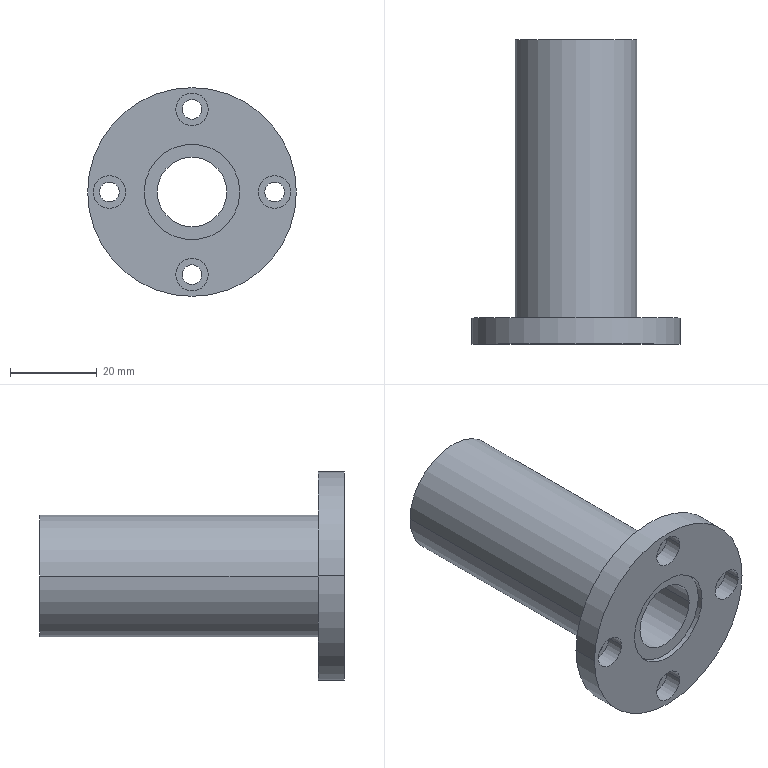Component | SolidWorks | SL021-1RoundFlangeExtendedType-416.SL4PRT-4 | 1 solid | 35 faces | box 48 x 70 x 48 mm | volume 34916 mm3 | cylinder 26 | plane 9 | commonest cylinder face diameters 4.5 x8 7.5 x8 22 x4 28 x2 48 x2 16 x2 | material Q235
STEP:
#1=COLOUR_RGB('',0.7922,0.8196,0.9333);
#2=FILL_AREA_STYLE_COLOUR('',#1);
#3=FILL_AREA_STYLE('',(#2));
#4=SURFACE_STYLE_FILL_AREA(#3);
#5=SURFACE_SIDE_STYLE('',(#4));
#6=SURFACE_STYLE_USAGE(.BOTH.,#5);
#7=PRESENTATION_STYLE_ASSIGNMENT((#6));
#8=CARTESIAN_POINT('',(-2.762,-0.807,0.1426));
#9=VERTEX_POINT('',#8);
#10=CARTESIAN_POINT('',(-1.66,-0.807,0.1426));
#11=VERTEX_POINT('',#10);
#12=CARTESIAN_POINT('',(-2.211,-0.807,0.1426));
#13=DIRECTION('',(-0.,1.,-0.));
#14=DIRECTION('',(-1.,0.,0.));
#15=AXIS2_PLACEMENT_3D('',#12,#13,#14);
#16=CIRCLE('',#15,0.5512);
#17=EDGE_CURVE('',#9,#11,#16,.T.);
#18=ORIENTED_EDGE('',*,*,#17,.T.);
#19=CARTESIAN_POINT('',(-1.66,1.713,0.1426));
#20=VERTEX_POINT('',#19);
#21=CARTESIAN_POINT('',(-1.66,1.713,0.1426));
#22=DIRECTION('',(-0.,1.,-0.));
#23=VECTOR('',#22,39.37);
#24=LINE('',#21,#23);
#25=EDGE_CURVE('',#11,#20,#24,.T.);
#26=ORIENTED_EDGE('',*,*,#25,.T.);
#27=CARTESIAN_POINT('',(-2.762,1.713,0.1426));
#28=VERTEX_POINT('',#27);
#29=CARTESIAN_POINT('',(-2.211,1.713,0.1426));
#30=DIRECTION('',(0.,-1.,0.));
#31=DIRECTION('',(-1.,0.,0.));
#32=AXIS2_PLACEMENT_3D('',#29,#30,#31);
#33=CIRCLE('',#32,0.5512);
#34=EDGE_CURVE('',#20,#28,#33,.T.);
#35=ORIENTED_EDGE('',*,*,#34,.T.);
#36=CARTESIAN_POINT('',(-2.762,1.713,0.1426));
#37=DIRECTION('',(-0.,1.,-0.));
#38=VECTOR('',#37,39.37);
#39=LINE('',#36,#38);
#40=EDGE_CURVE('',#9,#28,#39,.T.);
#41=ORIENTED_EDGE('',*,*,#40,.F.);
#42=EDGE_LOOP('',(#18,#26,#35,#41));
#43=FACE_OUTER_BOUND('',#42,.T.);
#44=CARTESIAN_POINT('',(-2.211,1.713,0.1426));
#45=DIRECTION('',(-0.,1.,-0.));
#46=DIRECTION('',(-1.,0.,0.));
#47=AXIS2_PLACEMENT_3D('',#44,#45,#46);
#48=CYLINDRICAL_SURFACE('',#47,0.5512);
#49=ADVANCED_FACE('',(#43),#48,.T.);
#50=CARTESIAN_POINT('',(-1.778,1.665,0.1426));
#51=VERTEX_POINT('',#50);
#52=CARTESIAN_POINT('',(-2.644,1.665,0.1426));
#53=VERTEX_POINT('',#52);
#54=CARTESIAN_POINT('',(-2.211,1.665,0.1426));
#55=DIRECTION('',(-0.,1.,-0.));
#56=DIRECTION('',(-1.,0.,0.));
#57=AXIS2_PLACEMENT_3D('',#54,#55,#56);
#58=CIRCLE('',#57,0.4331);
#59=EDGE_CURVE('',#51,#53,#58,.T.);
#60=ORIENTED_EDGE('',*,*,#59,.F.);
#61=CARTESIAN_POINT('',(-1.778,1.713,0.1426));
#62=VERTEX_POINT('',#61);
#63=CARTESIAN_POINT('',(-1.778,1.713,0.1426));
#64=DIRECTION('',(-0.,1.,-0.));
#65=VECTOR('',#64,39.37);
#66=LINE('',#63,#65);
#67=EDGE_CURVE('',#51,#62,#66,.T.);
#68=ORIENTED_EDGE('',*,*,#67,.T.);
#69=CARTESIAN_POINT('',(-2.644,1.713,0.1426));
#70=VERTEX_POINT('',#69);
#71=CARTESIAN_POINT('',(-2.211,1.713,0.1426));
#72=DIRECTION('',(0.,-1.,0.));
#73=DIRECTION('',(-1.,0.,0.));
#74=AXIS2_PLACEMENT_3D('',#71,#72,#73);
#75=CIRCLE('',#74,0.4331);
#76=EDGE_CURVE('',#70,#62,#75,.T.);
#77=ORIENTED_EDGE('',*,*,#76,.F.);
#78=CARTESIAN_POINT('',(-2.644,1.713,0.1426));
#79=DIRECTION('',(-0.,1.,-0.));
#80=VECTOR('',#79,39.37);
#81=LINE('',#78,#80);
#82=EDGE_CURVE('',#53,#70,#81,.T.);
#83=ORIENTED_EDGE('',*,*,#82,.F.);
#84=EDGE_LOOP('',(#60,#68,#77,#83));
#85=FACE_OUTER_BOUND('',#84,.T.);
#86=CARTESIAN_POINT('',(-2.211,1.713,0.1426));
#87=DIRECTION('',(-0.,1.,-0.));
#88=DIRECTION('',(-1.,0.,0.));
#89=AXIS2_PLACEMENT_3D('',#86,#87,#88);
#90=CYLINDRICAL_SURFACE('',#89,0.4331);
#91=ADVANCED_FACE('',(#85),#90,.F.);
#92=CARTESIAN_POINT('',(-3.156,-1.043,0.1426));
#93=VERTEX_POINT('',#92);
#94=CARTESIAN_POINT('',(-1.266,-1.043,0.1426));
#95=VERTEX_POINT('',#94);
#96=CARTESIAN_POINT('',(-2.211,-1.043,0.1426));
#97=DIRECTION('',(-0.,1.,-0.));
#98=DIRECTION('',(-1.,0.,0.));
#99=AXIS2_PLACEMENT_3D('',#96,#97,#98);
#100=CIRCLE('',#99,0.9449);
#101=EDGE_CURVE('',#93,#95,#100,.T.);
#102=ORIENTED_EDGE('',*,*,#101,.T.);
#103=CARTESIAN_POINT('',(-1.266,-0.807,0.1426));
#104=VERTEX_POINT('',#103);
#105=CARTESIAN_POINT('',(-1.266,1.713,0.1426));
#106=DIRECTION('',(-0.,1.,-0.));
#107=VECTOR('',#106,39.37);
#108=LINE('',#105,#107);
#109=EDGE_CURVE('',#95,#104,#108,.T.);
#110=ORIENTED_EDGE('',*,*,#109,.T.);
#111=CARTESIAN_POINT('',(-3.156,-0.807,0.1426));
#112=VERTEX_POINT('',#111);
#113=CARTESIAN_POINT('',(-2.211,-0.807,0.1426));
#114=DIRECTION('',(-0.,1.,-0.));
#115=DIRECTION('',(-1.,0.,0.));
#116=AXIS2_PLACEMENT_3D('',#113,#114,#115);
#117=CIRCLE('',#116,0.9449);
#118=EDGE_CURVE('',#112,#104,#117,.T.);
#119=ORIENTED_EDGE('',*,*,#118,.F.);
#120=CARTESIAN_POINT('',(-3.156,1.713,0.1426));
#121=DIRECTION('',(-0.,1.,-0.));
#122=VECTOR('',#121,39.37);
#123=LINE('',#120,#122);
#124=EDGE_CURVE('',#93,#112,#123,.T.);
#125=ORIENTED_EDGE('',*,*,#124,.F.);
#126=EDGE_LOOP('',(#102,#110,#119,#125));
#127=FACE_OUTER_BOUND('',#126,.T.);
#128=CARTESIAN_POINT('',(-2.211,1.713,0.1426));
#129=DIRECTION('',(-0.,1.,-0.));
#130=DIRECTION('',(-1.,0.,0.));
#131=AXIS2_PLACEMENT_3D('',#128,#129,#130);
#132=CYLINDRICAL_SURFACE('',#131,0.9449);
#133=ADVANCED_FACE('',(#127),#132,.T.);
#134=CARTESIAN_POINT('',(-2.3,-0.807,0.8906));
#135=VERTEX_POINT('',#134);
#136=CARTESIAN_POINT('',(-2.123,-0.807,0.8906));
#137=VERTEX_POINT('',#136);
#138=CARTESIAN_POINT('',(-2.211,-0.807,0.8906));
#139=DIRECTION('',(0.,-1.,0.));
#140=DIRECTION('',(1.,0.,0.));
#141=AXIS2_PLACEMENT_3D('',#138,#139,#140);
#142=CIRCLE('',#141,0.08858);
#143=EDGE_CURVE('',#135,#137,#142,.T.);
#144=ORIENTED_EDGE('',*,*,#143,.F.);
#145=CARTESIAN_POINT('',(-2.3,-0.8819,0.8906));
#146=VERTEX_POINT('',#145);
#147=CARTESIAN_POINT('',(-2.3,1.713,0.8906));
#148=DIRECTION('',(0.,-1.,0.));
#149=VECTOR('',#148,39.37);
#150=LINE('',#147,#149);
#151=EDGE_CURVE('',#135,#146,#150,.T.);
#152=ORIENTED_EDGE('',*,*,#151,.T.);
#153=CARTESIAN_POINT('',(-2.123,-0.8819,0.8906));
#154=VERTEX_POINT('',#153);
#155=CARTESIAN_POINT('',(-2.211,-0.8819,0.8906));
#156=DIRECTION('',(-0.,1.,-0.));
#157=DIRECTION('',(1.,0.,0.));
#158=AXIS2_PLACEMENT_3D('',#155,#156,#157);
#159=CIRCLE('',#158,0.08858);
#160=EDGE_CURVE('',#154,#146,#159,.T.);
#161=ORIENTED_EDGE('',*,*,#160,.F.);
#162=CARTESIAN_POINT('',(-2.123,1.713,0.8906));
#163=DIRECTION('',(0.,-1.,0.));
#164=VECTOR('',#163,39.37);
#165=LINE('',#162,#164);
#166=EDGE_CURVE('',#137,#154,#165,.T.);
#167=ORIENTED_EDGE('',*,*,#166,.F.);
#168=EDGE_LOOP('',(#144,#152,#161,#167));
#169=FACE_OUTER_BOUND('',#168,.T.);
#170=CARTESIAN_POINT('',(-2.211,1.713,0.8906));
#171=DIRECTION('',(0.,-1.,0.));
#172=DIRECTION('',(1.,0.,0.));
#173=AXIS2_PLACEMENT_3D('',#170,#171,#172);
#174=CYLINDRICAL_SURFACE('',#173,0.08858);
#175=ADVANCED_FACE('',(#169),#174,.F.);
#176=CARTESIAN_POINT('',(-1.552,-0.807,0.1426));
#177=VERTEX_POINT('',#176);
#178=CARTESIAN_POINT('',(-1.375,-0.807,0.1426));
#179=VERTEX_POINT('',#178);
#180=CARTESIAN_POINT('',(-1.463,-0.807,0.1426));
#181=DIRECTION('',(0.,-1.,0.));
#182=DIRECTION('',(1.,0.,-0.));
#183=AXIS2_PLACEMENT_3D('',#180,#181,#182);
#184=CIRCLE('',#183,0.08858);
#185=EDGE_CURVE('',#177,#179,#184,.T.);
#186=ORIENTED_EDGE('',*,*,#185,.F.);
#187=CARTESIAN_POINT('',(-1.552,-0.8819,0.1426));
#188=VERTEX_POINT('',#187);
#189=CARTESIAN_POINT('',(-1.552,1.713,0.1426));
#190=DIRECTION('',(0.,-1.,0.));
#191=VECTOR('',#190,39.37);
#192=LINE('',#189,#191);
#193=EDGE_CURVE('',#177,#188,#192,.T.);
#194=ORIENTED_EDGE('',*,*,#193,.T.);
#195=CARTESIAN_POINT('',(-1.375,-0.8819,0.1426));
#196=VERTEX_POINT('',#195);
#197=CARTESIAN_POINT('',(-1.463,-0.8819,0.1426));
#198=DIRECTION('',(-0.,1.,-0.));
#199=DIRECTION('',(1.,0.,-0.));
#200=AXIS2_PLACEMENT_3D('',#197,#198,#199);
#201=CIRCLE('',#200,0.08858);
#202=EDGE_CURVE('',#196,#188,#201,.T.);
#203=ORIENTED_EDGE('',*,*,#202,.F.);
#204=CARTESIAN_POINT('',(-1.375,1.713,0.1426));
#205=DIRECTION('',(0.,-1.,0.));
#206=VECTOR('',#205,39.37);
#207=LINE('',#204,#206);
#208=EDGE_CURVE('',#179,#196,#207,.T.);
#209=ORIENTED_EDGE('',*,*,#208,.F.);
#210=EDGE_LOOP('',(#186,#194,#203,#209));
#211=FACE_OUTER_BOUND('',#210,.T.);
#212=CARTESIAN_POINT('',(-1.463,1.713,0.1426));
#213=DIRECTION('',(0.,-1.,0.));
#214=DIRECTION('',(1.,0.,-0.));
#215=AXIS2_PLACEMENT_3D('',#212,#213,#214);
#216=CYLINDRICAL_SURFACE('',#215,0.08858);
#217=ADVANCED_FACE('',(#211),#216,.F.);
#218=CARTESIAN_POINT('',(-2.3,-0.807,-0.6054));
#219=VERTEX_POINT('',#218);
#220=CARTESIAN_POINT('',(-2.123,-0.807,-0.6054));
#221=VERTEX_POINT('',#220);
#222=CARTESIAN_POINT('',(-2.211,-0.807,-0.6054));
#223=DIRECTION('',(0.,-1.,0.));
#224=DIRECTION('',(1.,0.,0.));
#225=AXIS2_PLACEMENT_3D('',#222,#223,#224);
#226=CIRCLE('',#225,0.08858);
#227=EDGE_CURVE('',#219,#221,#226,.T.);
#228=ORIENTED_EDGE('',*,*,#227,.F.);
#229=CARTESIAN_POINT('',(-2.3,-0.8819,-0.6054));
#230=VERTEX_POINT('',#229);
#231=CARTESIAN_POINT('',(-2.3,1.713,-0.6054));
#232=DIRECTION('',(0.,-1.,0.));
#233=VECTOR('',#232,39.37);
#234=LINE('',#231,#233);
#235=EDGE_CURVE('',#219,#230,#234,.T.);
#236=ORIENTED_EDGE('',*,*,#235,.T.);
#237=CARTESIAN_POINT('',(-2.123,-0.8819,-0.6054));
#238=VERTEX_POINT('',#237);
#239=CARTESIAN_POINT('',(-2.211,-0.8819,-0.6054));
#240=DIRECTION('',(-0.,1.,-0.));
#241=DIRECTION('',(1.,0.,0.));
#242=AXIS2_PLACEMENT_3D('',#239,#240,#241);
#243=CIRCLE('',#242,0.08858);
#244=EDGE_CURVE('',#238,#230,#243,.T.);
#245=ORIENTED_EDGE('',*,*,#244,.F.);
#246=CARTESIAN_POINT('',(-2.123,1.713,-0.6054));
#247=DIRECTION('',(0.,-1.,0.));
#248=VECTOR('',#247,39.37);
#249=LINE('',#246,#248);
#250=EDGE_CURVE('',#221,#238,#249,.T.);
#251=ORIENTED_EDGE('',*,*,#250,.F.);
#252=EDGE_LOOP('',(#228,#236,#245,#251));
#253=FACE_OUTER_BOUND('',#252,.T.);
#254=CARTESIAN_POINT('',(-2.211,1.713,-0.6054));
#255=DIRECTION('',(0.,-1.,0.));
#256=DIRECTION('',(1.,0.,0.));
#257=AXIS2_PLACEMENT_3D('',#254,#255,#256);
#258=CYLINDRICAL_SURFACE('',#257,0.08858);
#259=ADVANCED_FACE('',(#253),#258,.F.);
#260=CARTESIAN_POINT('',(-3.048,-0.807,0.1426));
#261=VERTEX_POINT('',#260);
#262=CARTESIAN_POINT('',(-2.871,-0.807,0.1426));
#263=VERTEX_POINT('',#262);
#264=CARTESIAN_POINT('',(-2.959,-0.807,0.1426));
#265=DIRECTION('',(0.,-1.,0.));
#266=DIRECTION('',(1.,0.,-0.));
#267=AXIS2_PLACEMENT_3D('',#264,#265,#266);
#268=CIRCLE('',#267,0.08858);
#269=EDGE_CURVE('',#261,#263,#268,.T.);
#270=ORIENTED_EDGE('',*,*,#269,.F.);
#271=CARTESIAN_POINT('',(-3.048,-0.8819,0.1426));
#272=VERTEX_POINT('',#271);
#273=CARTESIAN_POINT('',(-3.048,1.713,0.1426));
#274=DIRECTION('',(0.,-1.,0.));
#275=VECTOR('',#274,39.37);
#276=LINE('',#273,#275);
#277=EDGE_CURVE('',#261,#272,#276,.T.);
#278=ORIENTED_EDGE('',*,*,#277,.T.);
#279=CARTESIAN_POINT('',(-2.871,-0.8819,0.1426));
#280=VERTEX_POINT('',#279);
#281=CARTESIAN_POINT('',(-2.959,-0.8819,0.1426));
#282=DIRECTION('',(-0.,1.,-0.));
#283=DIRECTION('',(1.,0.,-0.));
#284=AXIS2_PLACEMENT_3D('',#281,#282,#283);
#285=CIRCLE('',#284,0.08858);
#286=EDGE_CURVE('',#280,#272,#285,.T.);
#287=ORIENTED_EDGE('',*,*,#286,.F.);
#288=CARTESIAN_POINT('',(-2.871,1.713,0.1426));
#289=DIRECTION('',(0.,-1.,0.));
#290=VECTOR('',#289,39.37);
#291=LINE('',#288,#290);
#292=EDGE_CURVE('',#263,#280,#291,.T.);
#293=ORIENTED_EDGE('',*,*,#292,.F.);
#294=EDGE_LOOP('',(#270,#278,#287,#293));
#295=FACE_OUTER_BOUND('',#294,.T.);
#296=CARTESIAN_POINT('',(-2.959,1.713,0.1426));
#297=DIRECTION('',(0.,-1.,0.));
#298=DIRECTION('',(1.,0.,-0.));
#299=AXIS2_PLACEMENT_3D('',#296,#297,#298);
#300=CYLINDRICAL_SURFACE('',#299,0.08858);
#301=ADVANCED_FACE('',(#295),#300,.F.);
#302=CARTESIAN_POINT('',(-1.896,-0.996,0.1426));
#303=VERTEX_POINT('',#302);
#304=CARTESIAN_POINT('',(-2.526,-0.996,0.1426));
#305=VERTEX_POINT('',#304);
#306=CARTESIAN_POINT('',(-2.211,-0.996,0.1426));
#307=DIRECTION('',(-0.,1.,-0.));
#308=DIRECTION('',(-1.,0.,0.));
#309=AXIS2_PLACEMENT_3D('',#306,#307,#308);
#310=CIRCLE('',#309,0.315);
#311=EDGE_CURVE('',#303,#305,#310,.T.);
#312=ORIENTED_EDGE('',*,*,#311,.F.);
#313=CARTESIAN_POINT('',(-1.896,1.665,0.1426));
#314=VERTEX_POINT('',#313);
#315=CARTESIAN_POINT('',(-1.896,1.713,0.1426));
#316=DIRECTION('',(-0.,1.,-0.));
#317=VECTOR('',#316,39.37);
#318=LINE('',#315,#317);
#319=EDGE_CURVE('',#303,#314,#318,.T.);
#320=ORIENTED_EDGE('',*,*,#319,.T.);
#321=CARTESIAN_POINT('',(-2.526,1.665,0.1426));
#322=VERTEX_POINT('',#321);
#323=CARTESIAN_POINT('',(-2.211,1.665,0.1426));
#324=DIRECTION('',(-0.,1.,-0.));
#325=DIRECTION('',(-1.,0.,0.));
#326=AXIS2_PLACEMENT_3D('',#323,#324,#325);
#327=CIRCLE('',#326,0.315);
#328=EDGE_CURVE('',#314,#322,#327,.T.);
#329=ORIENTED_EDGE('',*,*,#328,.T.);
#330=CARTESIAN_POINT('',(-2.526,1.713,0.1426));
#331=DIRECTION('',(-0.,1.,-0.));
#332=VECTOR('',#331,39.37);
#333=LINE('',#330,#332);
#334=EDGE_CURVE('',#305,#322,#333,.T.);
#335=ORIENTED_EDGE('',*,*,#334,.F.);
#336=EDGE_LOOP('',(#312,#320,#329,#335));
#337=FACE_OUTER_BOUND('',#336,.T.);
#338=CARTESIAN_POINT('',(-2.211,1.713,0.1426));
#339=DIRECTION('',(-0.,1.,-0.));
#340=DIRECTION('',(-1.,0.,0.));
#341=AXIS2_PLACEMENT_3D('',#338,#339,#340);
#342=CYLINDRICAL_SURFACE('',#341,0.315);
#343=ADVANCED_FACE('',(#337),#342,.F.);
#344=CARTESIAN_POINT('',(-1.778,-1.043,0.1426));
#345=VERTEX_POINT('',#344);
#346=CARTESIAN_POINT('',(-2.644,-1.043,0.1426));
#347=VERTEX_POINT('',#346);
#348=CARTESIAN_POINT('',(-2.211,-1.043,0.1426));
#349=DIRECTION('',(-0.,1.,-0.));
#350=DIRECTION('',(-1.,0.,0.));
#351=AXIS2_PLACEMENT_3D('',#348,#349,#350);
#352=CIRCLE('',#351,0.4331);
#353=EDGE_CURVE('',#345,#347,#352,.T.);
#354=ORIENTED_EDGE('',*,*,#353,.F.);
#355=CARTESIAN_POINT('',(-1.778,-0.996,0.1426));
#356=VERTEX_POINT('',#355);
#357=CARTESIAN_POINT('',(-1.778,1.713,0.1426));
#358=DIRECTION('',(-0.,1.,-0.));
#359=VECTOR('',#358,39.37);
#360=LINE('',#357,#359);
#361=EDGE_CURVE('',#345,#356,#360,.T.);
#362=ORIENTED_EDGE('',*,*,#361,.T.);
#363=CARTESIAN_POINT('',(-2.644,-0.996,0.1426));
#364=VERTEX_POINT('',#363);
#365=CARTESIAN_POINT('',(-2.211,-0.996,0.1426));
#366=DIRECTION('',(0.,-1.,0.));
#367=DIRECTION('',(-1.,0.,0.));
#368=AXIS2_PLACEMENT_3D('',#365,#366,#367);
#369=CIRCLE('',#368,0.4331);
#370=EDGE_CURVE('',#364,#356,#369,.T.);
#371=ORIENTED_EDGE('',*,*,#370,.F.);
#372=CARTESIAN_POINT('',(-2.644,1.713,0.1426));
#373=DIRECTION('',(-0.,1.,-0.));
#374=VECTOR('',#373,39.37);
#375=LINE('',#372,#374);
#376=EDGE_CURVE('',#347,#364,#375,.T.);
#377=ORIENTED_EDGE('',*,*,#376,.F.);
#378=EDGE_LOOP('',(#354,#362,#371,#377));
#379=FACE_OUTER_BOUND('',#378,.T.);
#380=CARTESIAN_POINT('',(-2.211,1.713,0.1426));
#381=DIRECTION('',(-0.,1.,-0.));
#382=DIRECTION('',(-1.,0.,0.));
#383=AXIS2_PLACEMENT_3D('',#380,#381,#382);
#384=CYLINDRICAL_SURFACE('',#383,0.4331);
#385=ADVANCED_FACE('',(#379),#384,.F.);
#386=CARTESIAN_POINT('',(-2.359,-0.8819,0.8906));
#387=VERTEX_POINT('',#386);
#388=CARTESIAN_POINT('',(-2.064,-0.8819,0.8906));
#389=VERTEX_POINT('',#388);
#390=CARTESIAN_POINT('',(-2.211,-0.8819,0.8906));
#391=DIRECTION('',(0.,-1.,0.));
#392=DIRECTION('',(1.,0.,0.));
#393=AXIS2_PLACEMENT_3D('',#390,#391,#392);
#394=CIRCLE('',#393,0.1476);
#395=EDGE_CURVE('',#387,#389,#394,.T.);
#396=ORIENTED_EDGE('',*,*,#395,.F.);
#397=CARTESIAN_POINT('',(-2.359,-1.043,0.8906));
#398=VERTEX_POINT('',#397);
#399=CARTESIAN_POINT('',(-2.359,-0.8819,0.8906));
#400=DIRECTION('',(0.,-1.,0.));
#401=VECTOR('',#400,39.37);
#402=LINE('',#399,#401);
#403=EDGE_CURVE('',#387,#398,#402,.T.);
#404=ORIENTED_EDGE('',*,*,#403,.T.);
#405=CARTESIAN_POINT('',(-2.064,-1.043,0.8906));
#406=VERTEX_POINT('',#405);
#407=CARTESIAN_POINT('',(-2.211,-1.043,0.8906));
#408=DIRECTION('',(-0.,1.,-0.));
#409=DIRECTION('',(1.,0.,0.));
#410=AXIS2_PLACEMENT_3D('',#407,#408,#409);
#411=CIRCLE('',#410,0.1476);
#412=EDGE_CURVE('',#406,#398,#411,.T.);
#413=ORIENTED_EDGE('',*,*,#412,.F.);
#414=CARTESIAN_POINT('',(-2.064,-0.8819,0.8906));
#415=DIRECTION('',(0.,-1.,0.));
#416=VECTOR('',#415,39.37);
#417=LINE('',#414,#416);
#418=EDGE_CURVE('',#389,#406,#417,.T.);
#419=ORIENTED_EDGE('',*,*,#418,.F.);
#420=EDGE_LOOP('',(#396,#404,#413,#419));
#421=FACE_OUTER_BOUND('',#420,.T.);
#422=CARTESIAN_POINT('',(-2.211,-0.8819,0.8906));
#423=DIRECTION('',(0.,-1.,0.));
#424=DIRECTION('',(1.,0.,0.));
#425=AXIS2_PLACEMENT_3D('',#422,#423,#424);
#426=CYLINDRICAL_SURFACE('',#425,0.1476);
#427=ADVANCED_FACE('',(#421),#426,.F.);
#428=CARTESIAN_POINT('',(-1.611,-0.8819,0.1426));
#429=VERTEX_POINT('',#428);
#430=CARTESIAN_POINT('',(-1.315,-0.8819,0.1426));
#431=VERTEX_POINT('',#430);
#432=CARTESIAN_POINT('',(-1.463,-0.8819,0.1426));
#433=DIRECTION('',(0.,-1.,0.));
#434=DIRECTION('',(1.,0.,-0.));
#435=AXIS2_PLACEMENT_3D('',#432,#433,#434);
#436=CIRCLE('',#435,0.1476);
#437=EDGE_CURVE('',#429,#431,#436,.T.);
#438=ORIENTED_EDGE('',*,*,#437,.F.);
#439=CARTESIAN_POINT('',(-1.611,-1.043,0.1426));
#440=VERTEX_POINT('',#439);
#441=CARTESIAN_POINT('',(-1.611,-0.8819,0.1426));
#442=DIRECTION('',(0.,-1.,0.));
#443=VECTOR('',#442,39.37);
#444=LINE('',#441,#443);
#445=EDGE_CURVE('',#429,#440,#444,.T.);
#446=ORIENTED_EDGE('',*,*,#445,.T.);
#447=CARTESIAN_POINT('',(-1.315,-1.043,0.1426));
#448=VERTEX_POINT('',#447);
#449=CARTESIAN_POINT('',(-1.463,-1.043,0.1426));
#450=DIRECTION('',(-0.,1.,-0.));
#451=DIRECTION('',(1.,0.,-0.));
#452=AXIS2_PLACEMENT_3D('',#449,#450,#451);
#453=CIRCLE('',#452,0.1476);
#454=EDGE_CURVE('',#448,#440,#453,.T.);
#455=ORIENTED_EDGE('',*,*,#454,.F.);
#456=CARTESIAN_POINT('',(-1.315,-0.8819,0.1426));
#457=DIRECTION('',(0.,-1.,0.));
#458=VECTOR('',#457,39.37);
#459=LINE('',#456,#458);
#460=EDGE_CURVE('',#431,#448,#459,.T.);
#461=ORIENTED_EDGE('',*,*,#460,.F.);
#462=EDGE_LOOP('',(#438,#446,#455,#461));
#463=FACE_OUTER_BOUND('',#462,.T.);
#464=CARTESIAN_POINT('',(-1.463,-0.8819,0.1426));
#465=DIRECTION('',(0.,-1.,0.));
#466=DIRECTION('',(1.,0.,-0.));
#467=AXIS2_PLACEMENT_3D('',#464,#465,#466);
#468=CYLINDRICAL_SURFACE('',#467,0.1476);
#469=ADVANCED_FACE('',(#463),#468,.F.);
#470=CARTESIAN_POINT('',(-2.359,-0.8819,-0.6054));
#471=VERTEX_POINT('',#470);
#472=CARTESIAN_POINT('',(-2.064,-0.8819,-0.6054));
#473=VERTEX_POINT('',#472);
#474=CARTESIAN_POINT('',(-2.211,-0.8819,-0.6054));
#475=DIRECTION('',(0.,-1.,0.));
#476=DIRECTION('',(1.,0.,0.));
#477=AXIS2_PLACEMENT_3D('',#474,#475,#476);
#478=CIRCLE('',#477,0.1476);
#479=EDGE_CURVE('',#471,#473,#478,.T.);
#480=ORIENTED_EDGE('',*,*,#479,.F.);
#481=CARTESIAN_POINT('',(-2.359,-1.043,-0.6054));
#482=VERTEX_POINT('',#481);
#483=CARTESIAN_POINT('',(-2.359,-0.8819,-0.6054));
#484=DIRECTION('',(0.,-1.,0.));
#485=VECTOR('',#484,39.37);
#486=LINE('',#483,#485);
#487=EDGE_CURVE('',#471,#482,#486,.T.);
#488=ORIENTED_EDGE('',*,*,#487,.T.);
#489=CARTESIAN_POINT('',(-2.064,-1.043,-0.6054));
#490=VERTEX_POINT('',#489);
#491=CARTESIAN_POINT('',(-2.211,-1.043,-0.6054));
#492=DIRECTION('',(-0.,1.,-0.));
#493=DIRECTION('',(1.,0.,0.));
#494=AXIS2_PLACEMENT_3D('',#491,#492,#493);
#495=CIRCLE('',#494,0.1476);
#496=EDGE_CURVE('',#490,#482,#495,.T.);
#497=ORIENTED_EDGE('',*,*,#496,.F.);
#498=CARTESIAN_POINT('',(-2.064,-0.8819,-0.6054));
#499=DIRECTION('',(0.,-1.,0.));
#500=VECTOR('',#499,39.37);
#501=LINE('',#498,#500);
#502=EDGE_CURVE('',#473,#490,#501,.T.);
#503=ORIENTED_EDGE('',*,*,#502,.F.);
#504=EDGE_LOOP('',(#480,#488,#497,#503));
#505=FACE_OUTER_BOUND('',#504,.T.);
#506=CARTESIAN_POINT('',(-2.211,-0.8819,-0.6054));
#507=DIRECTION('',(0.,-1.,0.));
#508=DIRECTION('',(1.,0.,0.));
#509=AXIS2_PLACEMENT_3D('',#506,#507,#508);
#510=CYLINDRICAL_SURFACE('',#509,0.1476);
#511=ADVANCED_FACE('',(#505),#510,.F.);
#512=CARTESIAN_POINT('',(-3.107,-0.8819,0.1426));
#513=VERTEX_POINT('',#512);
#514=CARTESIAN_POINT('',(-2.812,-0.8819,0.1426));
#515=VERTEX_POINT('',#514);
#516=CARTESIAN_POINT('',(-2.959,-0.8819,0.1426));
#517=DIRECTION('',(0.,-1.,0.));
#518=DIRECTION('',(1.,0.,-0.));
#519=AXIS2_PLACEMENT_3D('',#516,#517,#518);
#520=CIRCLE('',#519,0.1476);
#521=EDGE_CURVE('',#513,#515,#520,.T.);
#522=ORIENTED_EDGE('',*,*,#521,.F.);
#523=CARTESIAN_POINT('',(-3.107,-1.043,0.1426));
#524=VERTEX_POINT('',#523);
#525=CARTESIAN_POINT('',(-3.107,-0.8819,0.1426));
#526=DIRECTION('',(0.,-1.,0.));
#527=VECTOR('',#526,39.37);
#528=LINE('',#525,#527);
#529=EDGE_CURVE('',#513,#524,#528,.T.);
#530=ORIENTED_EDGE('',*,*,#529,.T.);
#531=CARTESIAN_POINT('',(-2.812,-1.043,0.1426));
#532=VERTEX_POINT('',#531);
#533=CARTESIAN_POINT('',(-2.959,-1.043,0.1426));
#534=DIRECTION('',(-0.,1.,-0.));
#535=DIRECTION('',(1.,0.,-0.));
#536=AXIS2_PLACEMENT_3D('',#533,#534,#535);
#537=CIRCLE('',#536,0.1476);
#538=EDGE_CURVE('',#532,#524,#537,.T.);
#539=ORIENTED_EDGE('',*,*,#538,.F.);
#540=CARTESIAN_POINT('',(-2.812,-0.8819,0.1426));
#541=DIRECTION('',(0.,-1.,0.));
#542=VECTOR('',#541,39.37);
#543=LINE('',#540,#542);
#544=EDGE_CURVE('',#515,#532,#543,.T.);
#545=ORIENTED_EDGE('',*,*,#544,.F.);
#546=EDGE_LOOP('',(#522,#530,#539,#545));
#547=FACE_OUTER_BOUND('',#546,.T.);
#548=CARTESIAN_POINT('',(-2.959,-0.8819,0.1426));
#549=DIRECTION('',(0.,-1.,0.));
#550=DIRECTION('',(1.,0.,-0.));
#551=AXIS2_PLACEMENT_3D('',#548,#549,#550);
#552=CYLINDRICAL_SURFACE('',#551,0.1476);
#553=ADVANCED_FACE('',(#547),#552,.F.);
#554=ORIENTED_EDGE('',*,*,#25,.F.);
#555=CARTESIAN_POINT('',(-2.211,-0.807,0.1426));
#556=DIRECTION('',(-0.,1.,-0.));
#557=DIRECTION('',(-1.,0.,0.));
#558=AXIS2_PLACEMENT_3D('',#555,#556,#557);
#559=CIRCLE('',#558,0.5512);
#560=EDGE_CURVE('',#11,#9,#559,.T.);
#561=ORIENTED_EDGE('',*,*,#560,.T.);
#562=ORIENTED_EDGE('',*,*,#40,.T.);
#563=CARTESIAN_POINT('',(-2.211,1.713,0.1426));
#564=DIRECTION('',(0.,-1.,0.));
#565=DIRECTION('',(-1.,0.,0.));
#566=AXIS2_PLACEMENT_3D('',#563,#564,#565);
#567=CIRCLE('',#566,0.5512);
#568=EDGE_CURVE('',#28,#20,#567,.T.);
#569=ORIENTED_EDGE('',*,*,#568,.T.);
#570=EDGE_LOOP('',(#554,#561,#562,#569));
#571=FACE_OUTER_BOUND('',#570,.T.);
#572=CARTESIAN_POINT('',(-2.211,1.713,0.1426));
#573=DIRECTION('',(-0.,1.,-0.));
#574=DIRECTION('',(-1.,0.,0.));
#575=AXIS2_PLACEMENT_3D('',#572,#573,#574);
#576=CYLINDRICAL_SURFACE('',#575,0.5512);
#577=ADVANCED_FACE('',(#571),#576,.T.);
#578=ORIENTED_EDGE('',*,*,#76,.T.);
#579=CARTESIAN_POINT('',(-2.211,1.713,0.1426));
#580=DIRECTION('',(0.,-1.,0.));
#581=DIRECTION('',(-1.,0.,0.));
#582=AXIS2_PLACEMENT_3D('',#579,#580,#581);
#583=CIRCLE('',#582,0.4331);
#584=EDGE_CURVE('',#62,#70,#583,.T.);
#585=ORIENTED_EDGE('',*,*,#584,.T.);
#586=EDGE_LOOP('',(#578,#585));
#587=FACE_BOUND('',#586,.T.);
#588=ORIENTED_EDGE('',*,*,#568,.F.);
#589=ORIENTED_EDGE('',*,*,#34,.F.);
#590=EDGE_LOOP('',(#588,#589));
#591=FACE_OUTER_BOUND('',#590,.T.);
#592=CARTESIAN_POINT('',(-2.211,1.713,0.615));
#593=DIRECTION('',(-0.,1.,-0.));
#594=DIRECTION('',(-1.,-0.,0.));
#595=AXIS2_PLACEMENT_3D('',#592,#593,#594);
#596=PLANE('',#595);
#597=ADVANCED_FACE('',(#587,#591),#596,.T.);
#598=ORIENTED_EDGE('',*,*,#17,.F.);
#599=ORIENTED_EDGE('',*,*,#560,.F.);
#600=EDGE_LOOP('',(#598,#599));
#601=FACE_BOUND('',#600,.T.);
#602=ORIENTED_EDGE('',*,*,#118,.T.);
#603=CARTESIAN_POINT('',(-2.211,-0.807,0.1426));
#604=DIRECTION('',(-0.,1.,-0.));
#605=DIRECTION('',(-1.,0.,0.));
#606=AXIS2_PLACEMENT_3D('',#603,#604,#605);
#607=CIRCLE('',#606,0.9449);
#608=EDGE_CURVE('',#104,#112,#607,.T.);
#609=ORIENTED_EDGE('',*,*,#608,.T.);
#610=EDGE_LOOP('',(#602,#609));
#611=FACE_OUTER_BOUND('',#610,.T.);
#612=CARTESIAN_POINT('',(-2.211,-0.807,0.8906));
#613=DIRECTION('',(0.,-1.,0.));
#614=DIRECTION('',(1.,0.,0.));
#615=AXIS2_PLACEMENT_3D('',#612,#613,#614);
#616=CIRCLE('',#615,0.08858);
#617=EDGE_CURVE('',#137,#135,#616,.T.);
#618=ORIENTED_EDGE('',*,*,#617,.T.);
#619=ORIENTED_EDGE('',*,*,#143,.T.);
#620=EDGE_LOOP('',(#618,#619));
#621=FACE_BOUND('',#620,.T.);
#622=CARTESIAN_POINT('',(-1.463,-0.807,0.1426));
#623=DIRECTION('',(0.,-1.,0.));
#624=DIRECTION('',(1.,0.,-0.));
#625=AXIS2_PLACEMENT_3D('',#622,#623,#624);
#626=CIRCLE('',#625,0.08858);
#627=EDGE_CURVE('',#179,#177,#626,.T.);
#628=ORIENTED_EDGE('',*,*,#627,.T.);
#629=ORIENTED_EDGE('',*,*,#185,.T.);
#630=EDGE_LOOP('',(#628,#629));
#631=FACE_BOUND('',#630,.T.);
#632=CARTESIAN_POINT('',(-2.211,-0.807,-0.6054));
#633=DIRECTION('',(0.,-1.,0.));
#634=DIRECTION('',(1.,0.,0.));
#635=AXIS2_PLACEMENT_3D('',#632,#633,#634);
#636=CIRCLE('',#635,0.08858);
#637=EDGE_CURVE('',#221,#219,#636,.T.);
#638=ORIENTED_EDGE('',*,*,#637,.T.);
#639=ORIENTED_EDGE('',*,*,#227,.T.);
#640=EDGE_LOOP('',(#638,#639));
#641=FACE_BOUND('',#640,.T.);
#642=CARTESIAN_POINT('',(-2.959,-0.807,0.1426));
#643=DIRECTION('',(0.,-1.,0.));
#644=DIRECTION('',(1.,0.,-0.));
#645=AXIS2_PLACEMENT_3D('',#642,#643,#644);
#646=CIRCLE('',#645,0.08858);
#647=EDGE_CURVE('',#263,#261,#646,.T.);
#648=ORIENTED_EDGE('',*,*,#647,.T.);
#649=ORIENTED_EDGE('',*,*,#269,.T.);
#650=EDGE_LOOP('',(#648,#649));
#651=FACE_BOUND('',#650,.T.);
#652=CARTESIAN_POINT('',(-2.211,-0.807,0.615));
#653=DIRECTION('',(-0.,1.,-0.));
#654=DIRECTION('',(-1.,-0.,0.));
#655=AXIS2_PLACEMENT_3D('',#652,#653,#654);
#656=PLANE('',#655);
#657=ADVANCED_FACE('',(#601,#611,#621,#631,#641,#651),#656,.T.);
#658=ORIENTED_EDGE('',*,*,#67,.F.);
#659=CARTESIAN_POINT('',(-2.211,1.665,0.1426));
#660=DIRECTION('',(-0.,1.,-0.));
#661=DIRECTION('',(-1.,0.,0.));
#662=AXIS2_PLACEMENT_3D('',#659,#660,#661);
#663=CIRCLE('',#662,0.4331);
#664=EDGE_CURVE('',#53,#51,#663,.T.);
#665=ORIENTED_EDGE('',*,*,#664,.F.);
#666=ORIENTED_EDGE('',*,*,#82,.T.);
#667=ORIENTED_EDGE('',*,*,#584,.F.);
#668=EDGE_LOOP('',(#658,#665,#666,#667));
#669=FACE_OUTER_BOUND('',#668,.T.);
#670=CARTESIAN_POINT('',(-2.211,1.713,0.1426));
#671=DIRECTION('',(-0.,1.,-0.));
#672=DIRECTION('',(-1.,0.,0.));
#673=AXIS2_PLACEMENT_3D('',#670,#671,#672);
#674=CYLINDRICAL_SURFACE('',#673,0.4331);
#675=ADVANCED_FACE('',(#669),#674,.F.);
#676=ORIENTED_EDGE('',*,*,#109,.F.);
#677=CARTESIAN_POINT('',(-2.211,-1.043,0.1426));
#678=DIRECTION('',(-0.,1.,-0.));
#679=DIRECTION('',(-1.,0.,0.));
#680=AXIS2_PLACEMENT_3D('',#677,#678,#679);
#681=CIRCLE('',#680,0.9449);
#682=EDGE_CURVE('',#95,#93,#681,.T.);
#683=ORIENTED_EDGE('',*,*,#682,.T.);
#684=ORIENTED_EDGE('',*,*,#124,.T.);
#685=ORIENTED_EDGE('',*,*,#608,.F.);
#686=EDGE_LOOP('',(#676,#683,#684,#685));
#687=FACE_OUTER_BOUND('',#686,.T.);
#688=CARTESIAN_POINT('',(-2.211,1.713,0.1426));
#689=DIRECTION('',(-0.,1.,-0.));
#690=DIRECTION('',(-1.,0.,0.));
#691=AXIS2_PLACEMENT_3D('',#688,#689,#690);
#692=CYLINDRICAL_SURFACE('',#691,0.9449);
#693=ADVANCED_FACE('',(#687),#692,.T.);
#694=ORIENTED_EDGE('',*,*,#151,.F.);
#695=ORIENTED_EDGE('',*,*,#617,.F.);
#696=ORIENTED_EDGE('',*,*,#166,.T.);
#697=CARTESIAN_POINT('',(-2.211,-0.8819,0.8906));
#698=DIRECTION('',(-0.,1.,-0.));
#699=DIRECTION('',(1.,0.,0.));
#700=AXIS2_PLACEMENT_3D('',#697,#698,#699);
#701=CIRCLE('',#700,0.08858);
#702=EDGE_CURVE('',#146,#154,#701,.T.);
#703=ORIENTED_EDGE('',*,*,#702,.F.);
#704=EDGE_LOOP('',(#694,#695,#696,#703));
#705=FACE_OUTER_BOUND('',#704,.T.);
#706=CARTESIAN_POINT('',(-2.211,1.713,0.8906));
#707=DIRECTION('',(0.,-1.,0.));
#708=DIRECTION('',(1.,0.,0.));
#709=AXIS2_PLACEMENT_3D('',#706,#707,#708);
#710=CYLINDRICAL_SURFACE('',#709,0.08858);
#711=ADVANCED_FACE('',(#705),#710,.F.);
#712=ORIENTED_EDGE('',*,*,#193,.F.);
#713=ORIENTED_EDGE('',*,*,#627,.F.);
#714=ORIENTED_EDGE('',*,*,#208,.T.);
#715=CARTESIAN_POINT('',(-1.463,-0.8819,0.1426));
#716=DIRECTION('',(-0.,1.,-0.));
#717=DIRECTION('',(1.,0.,-0.));
#718=AXIS2_PLACEMENT_3D('',#715,#716,#717);
#719=CIRCLE('',#718,0.08858);
#720=EDGE_CURVE('',#188,#196,#719,.T.);
#721=ORIENTED_EDGE('',*,*,#720,.F.);
#722=EDGE_LOOP('',(#712,#713,#714,#721));
#723=FACE_OUTER_BOUND('',#722,.T.);
#724=CARTESIAN_POINT('',(-1.463,1.713,0.1426));
#725=DIRECTION('',(0.,-1.,0.));
#726=DIRECTION('',(1.,0.,-0.));
#727=AXIS2_PLACEMENT_3D('',#724,#725,#726);
#728=CYLINDRICAL_SURFACE('',#727,0.08858);
#729=ADVANCED_FACE('',(#723),#728,.F.);
#730=ORIENTED_EDGE('',*,*,#235,.F.);
#731=ORIENTED_EDGE('',*,*,#637,.F.);
#732=ORIENTED_EDGE('',*,*,#250,.T.);
#733=CARTESIAN_POINT('',(-2.211,-0.8819,-0.6054));
#734=DIRECTION('',(-0.,1.,-0.));
#735=DIRECTION('',(1.,0.,0.));
#736=AXIS2_PLACEMENT_3D('',#733,#734,#735);
#737=CIRCLE('',#736,0.08858);
#738=EDGE_CURVE('',#230,#238,#737,.T.);
#739=ORIENTED_EDGE('',*,*,#738,.F.);
#740=EDGE_LOOP('',(#730,#731,#732,#739));
#741=FACE_OUTER_BOUND('',#740,.T.);
#742=CARTESIAN_POINT('',(-2.211,1.713,-0.6054));
#743=DIRECTION('',(0.,-1.,0.));
#744=DIRECTION('',(1.,0.,0.));
#745=AXIS2_PLACEMENT_3D('',#742,#743,#744);
#746=CYLINDRICAL_SURFACE('',#745,0.08858);
#747=ADVANCED_FACE('',(#741),#746,.F.);
#748=ORIENTED_EDGE('',*,*,#277,.F.);
#749=ORIENTED_EDGE('',*,*,#647,.F.);
#750=ORIENTED_EDGE('',*,*,#292,.T.);
#751=CARTESIAN_POINT('',(-2.959,-0.8819,0.1426));
#752=DIRECTION('',(-0.,1.,-0.));
#753=DIRECTION('',(1.,0.,-0.));
#754=AXIS2_PLACEMENT_3D('',#751,#752,#753);
#755=CIRCLE('',#754,0.08858);
#756=EDGE_CURVE('',#272,#280,#755,.T.);
#757=ORIENTED_EDGE('',*,*,#756,.F.);
#758=EDGE_LOOP('',(#748,#749,#750,#757));
#759=FACE_OUTER_BOUND('',#758,.T.);
#760=CARTESIAN_POINT('',(-2.959,1.713,0.1426));
#761=DIRECTION('',(0.,-1.,0.));
#762=DIRECTION('',(1.,0.,-0.));
#763=AXIS2_PLACEMENT_3D('',#760,#761,#762);
#764=CYLINDRICAL_SURFACE('',#763,0.08858);
#765=ADVANCED_FACE('',(#759),#764,.F.);
#766=ORIENTED_EDGE('',*,*,#664,.T.);
#767=ORIENTED_EDGE('',*,*,#59,.T.);
#768=EDGE_LOOP('',(#766,#767));
#769=FACE_OUTER_BOUND('',#768,.T.);
#770=CARTESIAN_POINT('',(-2.211,1.665,0.1426));
#771=DIRECTION('',(-0.,1.,-0.));
#772=DIRECTION('',(-1.,0.,0.));
#773=AXIS2_PLACEMENT_3D('',#770,#771,#772);
#774=CIRCLE('',#773,0.315);
#775=EDGE_CURVE('',#322,#314,#774,.T.);
#776=ORIENTED_EDGE('',*,*,#775,.F.);
#777=ORIENTED_EDGE('',*,*,#328,.F.);
#778=EDGE_LOOP('',(#776,#777));
#779=FACE_BOUND('',#778,.T.);
#780=CARTESIAN_POINT('',(-2.211,1.665,0.615));
#781=DIRECTION('',(0.,-1.,0.));
#782=DIRECTION('',(1.,0.,-0.));
#783=AXIS2_PLACEMENT_3D('',#780,#781,#782);
#784=PLANE('',#783);
#785=ADVANCED_FACE('',(#769,#779),#784,.F.);
#786=ORIENTED_EDGE('',*,*,#101,.F.);
#787=ORIENTED_EDGE('',*,*,#682,.F.);
#788=EDGE_LOOP('',(#786,#787));
#789=FACE_OUTER_BOUND('',#788,.T.);
#790=CARTESIAN_POINT('',(-2.211,-1.043,0.1426));
#791=DIRECTION('',(-0.,1.,-0.));
#792=DIRECTION('',(-1.,0.,0.));
#793=AXIS2_PLACEMENT_3D('',#790,#791,#792);
#794=CIRCLE('',#793,0.4331);
#795=EDGE_CURVE('',#347,#345,#794,.T.);
#796=ORIENTED_EDGE('',*,*,#795,.T.);
#797=ORIENTED_EDGE('',*,*,#353,.T.);
#798=EDGE_LOOP('',(#796,#797));
#799=FACE_BOUND('',#798,.T.);
#800=ORIENTED_EDGE('',*,*,#412,.T.);
#801=CARTESIAN_POINT('',(-2.211,-1.043,0.8906));
#802=DIRECTION('',(-0.,1.,-0.));
#803=DIRECTION('',(1.,0.,0.));
#804=AXIS2_PLACEMENT_3D('',#801,#802,#803);
#805=CIRCLE('',#804,0.1476);
#806=EDGE_CURVE('',#398,#406,#805,.T.);
#807=ORIENTED_EDGE('',*,*,#806,.T.);
#808=EDGE_LOOP('',(#800,#807));
#809=FACE_BOUND('',#808,.T.);
#810=ORIENTED_EDGE('',*,*,#454,.T.);
#811=CARTESIAN_POINT('',(-1.463,-1.043,0.1426));
#812=DIRECTION('',(-0.,1.,-0.));
#813=DIRECTION('',(1.,0.,-0.));
#814=AXIS2_PLACEMENT_3D('',#811,#812,#813);
#815=CIRCLE('',#814,0.1476);
#816=EDGE_CURVE('',#440,#448,#815,.T.);
#817=ORIENTED_EDGE('',*,*,#816,.T.);
#818=EDGE_LOOP('',(#810,#817));
#819=FACE_BOUND('',#818,.T.);
#820=ORIENTED_EDGE('',*,*,#496,.T.);
#821=CARTESIAN_POINT('',(-2.211,-1.043,-0.6054));
#822=DIRECTION('',(-0.,1.,-0.));
#823=DIRECTION('',(1.,0.,0.));
#824=AXIS2_PLACEMENT_3D('',#821,#822,#823);
#825=CIRCLE('',#824,0.1476);
#826=EDGE_CURVE('',#482,#490,#825,.T.);
#827=ORIENTED_EDGE('',*,*,#826,.T.);
#828=EDGE_LOOP('',(#820,#827));
#829=FACE_BOUND('',#828,.T.);
#830=ORIENTED_EDGE('',*,*,#538,.T.);
#831=CARTESIAN_POINT('',(-2.959,-1.043,0.1426));
#832=DIRECTION('',(-0.,1.,-0.));
#833=DIRECTION('',(1.,0.,-0.));
#834=AXIS2_PLACEMENT_3D('',#831,#832,#833);
#835=CIRCLE('',#834,0.1476);
#836=EDGE_CURVE('',#524,#532,#835,.T.);
#837=ORIENTED_EDGE('',*,*,#836,.T.);
#838=EDGE_LOOP('',(#830,#837));
#839=FACE_BOUND('',#838,.T.);
#840=CARTESIAN_POINT('',(-2.211,-1.043,0.615));
#841=DIRECTION('',(0.,-1.,0.));
#842=DIRECTION('',(1.,0.,-0.));
#843=AXIS2_PLACEMENT_3D('',#840,#841,#842);
#844=PLANE('',#843);
#845=ADVANCED_FACE('',(#789,#799,#809,#819,#829,#839),#844,.T.);
#846=ORIENTED_EDGE('',*,*,#160,.T.);
#847=ORIENTED_EDGE('',*,*,#702,.T.);
#848=EDGE_LOOP('',(#846,#847));
#849=FACE_BOUND('',#848,.T.);
#850=CARTESIAN_POINT('',(-2.211,-0.8819,0.8906));
#851=DIRECTION('',(0.,-1.,0.));
#852=DIRECTION('',(1.,0.,0.));
#853=AXIS2_PLACEMENT_3D('',#850,#851,#852);
#854=CIRCLE('',#853,0.1476);
#855=EDGE_CURVE('',#389,#387,#854,.T.);
#856=ORIENTED_EDGE('',*,*,#855,.T.);
#857=ORIENTED_EDGE('',*,*,#395,.T.);
#858=EDGE_LOOP('',(#856,#857));
#859=FACE_OUTER_BOUND('',#858,.T.);
#860=CARTESIAN_POINT('',(-2.211,-0.8819,0.8906));
#861=DIRECTION('',(0.,-1.,0.));
#862=DIRECTION('',(1.,0.,-0.));
#863=AXIS2_PLACEMENT_3D('',#860,#861,#862);
#864=PLANE('',#863);
#865=ADVANCED_FACE('',(#849,#859),#864,.T.);
#866=ORIENTED_EDGE('',*,*,#202,.T.);
#867=ORIENTED_EDGE('',*,*,#720,.T.);
#868=EDGE_LOOP('',(#866,#867));
#869=FACE_BOUND('',#868,.T.);
#870=CARTESIAN_POINT('',(-1.463,-0.8819,0.1426));
#871=DIRECTION('',(0.,-1.,0.));
#872=DIRECTION('',(1.,0.,-0.));
#873=AXIS2_PLACEMENT_3D('',#870,#871,#872);
#874=CIRCLE('',#873,0.1476);
#875=EDGE_CURVE('',#431,#429,#874,.T.);
#876=ORIENTED_EDGE('',*,*,#875,.T.);
#877=ORIENTED_EDGE('',*,*,#437,.T.);
#878=EDGE_LOOP('',(#876,#877));
#879=FACE_OUTER_BOUND('',#878,.T.);
#880=CARTESIAN_POINT('',(-1.463,-0.8819,0.1426));
#881=DIRECTION('',(0.,-1.,0.));
#882=DIRECTION('',(1.,0.,-0.));
#883=AXIS2_PLACEMENT_3D('',#880,#881,#882);
#884=PLANE('',#883);
#885=ADVANCED_FACE('',(#869,#879),#884,.T.);
#886=ORIENTED_EDGE('',*,*,#244,.T.);
#887=ORIENTED_EDGE('',*,*,#738,.T.);
#888=EDGE_LOOP('',(#886,#887));
#889=FACE_BOUND('',#888,.T.);
#890=CARTESIAN_POINT('',(-2.211,-0.8819,-0.6054));
#891=DIRECTION('',(0.,-1.,0.));
#892=DIRECTION('',(1.,0.,0.));
#893=AXIS2_PLACEMENT_3D('',#890,#891,#892);
#894=CIRCLE('',#893,0.1476);
#895=EDGE_CURVE('',#473,#471,#894,.T.);
#896=ORIENTED_EDGE('',*,*,#895,.T.);
#897=ORIENTED_EDGE('',*,*,#479,.T.);
#898=EDGE_LOOP('',(#896,#897));
#899=FACE_OUTER_BOUND('',#898,.T.);
#900=CARTESIAN_POINT('',(-2.211,-0.8819,-0.6054));
#901=DIRECTION('',(0.,-1.,0.));
#902=DIRECTION('',(1.,0.,-0.));
#903=AXIS2_PLACEMENT_3D('',#900,#901,#902);
#904=PLANE('',#903);
#905=ADVANCED_FACE('',(#889,#899),#904,.T.);
#906=ORIENTED_EDGE('',*,*,#286,.T.);
#907=ORIENTED_EDGE('',*,*,#756,.T.);
#908=EDGE_LOOP('',(#906,#907));
#909=FACE_BOUND('',#908,.T.);
#910=CARTESIAN_POINT('',(-2.959,-0.8819,0.1426));
#911=DIRECTION('',(0.,-1.,0.));
#912=DIRECTION('',(1.,0.,-0.));
#913=AXIS2_PLACEMENT_3D('',#910,#911,#912);
#914=CIRCLE('',#913,0.1476);
#915=EDGE_CURVE('',#515,#513,#914,.T.);
#916=ORIENTED_EDGE('',*,*,#915,.T.);
#917=ORIENTED_EDGE('',*,*,#521,.T.);
#918=EDGE_LOOP('',(#916,#917));
#919=FACE_OUTER_BOUND('',#918,.T.);
#920=CARTESIAN_POINT('',(-2.959,-0.8819,0.1426));
#921=DIRECTION('',(0.,-1.,0.));
#922=DIRECTION('',(1.,0.,-0.));
#923=AXIS2_PLACEMENT_3D('',#920,#921,#922);
#924=PLANE('',#923);
#925=ADVANCED_FACE('',(#909,#919),#924,.T.);
#926=ORIENTED_EDGE('',*,*,#319,.F.);
#927=CARTESIAN_POINT('',(-2.211,-0.996,0.1426));
#928=DIRECTION('',(-0.,1.,-0.));
#929=DIRECTION('',(-1.,0.,0.));
#930=AXIS2_PLACEMENT_3D('',#927,#928,#929);
#931=CIRCLE('',#930,0.315);
#932=EDGE_CURVE('',#305,#303,#931,.T.);
#933=ORIENTED_EDGE('',*,*,#932,.F.);
#934=ORIENTED_EDGE('',*,*,#334,.T.);
#935=ORIENTED_EDGE('',*,*,#775,.T.);
#936=EDGE_LOOP('',(#926,#933,#934,#935));
#937=FACE_OUTER_BOUND('',#936,.T.);
#938=CARTESIAN_POINT('',(-2.211,1.713,0.1426));
#939=DIRECTION('',(-0.,1.,-0.));
#940=DIRECTION('',(-1.,0.,0.));
#941=AXIS2_PLACEMENT_3D('',#938,#939,#940);
#942=CYLINDRICAL_SURFACE('',#941,0.315);
#943=ADVANCED_FACE('',(#937),#942,.F.);
#944=ORIENTED_EDGE('',*,*,#361,.F.);
#945=ORIENTED_EDGE('',*,*,#795,.F.);
#946=ORIENTED_EDGE('',*,*,#376,.T.);
#947=CARTESIAN_POINT('',(-2.211,-0.996,0.1426));
#948=DIRECTION('',(0.,-1.,0.));
#949=DIRECTION('',(-1.,0.,0.));
#950=AXIS2_PLACEMENT_3D('',#947,#948,#949);
#951=CIRCLE('',#950,0.4331);
#952=EDGE_CURVE('',#356,#364,#951,.T.);
#953=ORIENTED_EDGE('',*,*,#952,.F.);
#954=EDGE_LOOP('',(#944,#945,#946,#953));
#955=FACE_OUTER_BOUND('',#954,.T.);
#956=CARTESIAN_POINT('',(-2.211,1.713,0.1426));
#957=DIRECTION('',(-0.,1.,-0.));
#958=DIRECTION('',(-1.,0.,0.));
#959=AXIS2_PLACEMENT_3D('',#956,#957,#958);
#960=CYLINDRICAL_SURFACE('',#959,0.4331);
#961=ADVANCED_FACE('',(#955),#960,.F.);
#962=ORIENTED_EDGE('',*,*,#403,.F.);
#963=ORIENTED_EDGE('',*,*,#855,.F.);
#964=ORIENTED_EDGE('',*,*,#418,.T.);
#965=ORIENTED_EDGE('',*,*,#806,.F.);
#966=EDGE_LOOP('',(#962,#963,#964,#965));
#967=FACE_OUTER_BOUND('',#966,.T.);
#968=CARTESIAN_POINT('',(-2.211,-0.8819,0.8906));
#969=DIRECTION('',(0.,-1.,0.));
#970=DIRECTION('',(1.,0.,0.));
#971=AXIS2_PLACEMENT_3D('',#968,#969,#970);
#972=CYLINDRICAL_SURFACE('',#971,0.1476);
#973=ADVANCED_FACE('',(#967),#972,.F.);
#974=ORIENTED_EDGE('',*,*,#445,.F.);
#975=ORIENTED_EDGE('',*,*,#875,.F.);
#976=ORIENTED_EDGE('',*,*,#460,.T.);
#977=ORIENTED_EDGE('',*,*,#816,.F.);
#978=EDGE_LOOP('',(#974,#975,#976,#977));
#979=FACE_OUTER_BOUND('',#978,.T.);
#980=CARTESIAN_POINT('',(-1.463,-0.8819,0.1426));
#981=DIRECTION('',(0.,-1.,0.));
#982=DIRECTION('',(1.,0.,-0.));
#983=AXIS2_PLACEMENT_3D('',#980,#981,#982);
#984=CYLINDRICAL_SURFACE('',#983,0.1476);
#985=ADVANCED_FACE('',(#979),#984,.F.);
#986=ORIENTED_EDGE('',*,*,#487,.F.);
#987=ORIENTED_EDGE('',*,*,#895,.F.);
#988=ORIENTED_EDGE('',*,*,#502,.T.);
#989=ORIENTED_EDGE('',*,*,#826,.F.);
#990=EDGE_LOOP('',(#986,#987,#988,#989));
#991=FACE_OUTER_BOUND('',#990,.T.);
#992=CARTESIAN_POINT('',(-2.211,-0.8819,-0.6054));
#993=DIRECTION('',(0.,-1.,0.));
#994=DIRECTION('',(1.,0.,0.));
#995=AXIS2_PLACEMENT_3D('',#992,#993,#994);
#996=CYLINDRICAL_SURFACE('',#995,0.1476);
#997=ADVANCED_FACE('',(#991),#996,.F.);
#998=ORIENTED_EDGE('',*,*,#529,.F.);
#999=ORIENTED_EDGE('',*,*,#915,.F.);
#1000=ORIENTED_EDGE('',*,*,#544,.T.);
#1001=ORIENTED_EDGE('',*,*,#836,.F.);
#1002=EDGE_LOOP('',(#998,#999,#1000,#1001));
#1003=FACE_OUTER_BOUND('',#1002,.T.);
#1004=CARTESIAN_POINT('',(-2.959,-0.8819,0.1426));
#1005=DIRECTION('',(0.,-1.,0.));
#1006=DIRECTION('',(1.,0.,-0.));
#1007=AXIS2_PLACEMENT_3D('',#1004,#1005,#1006);
#1008=CYLINDRICAL_SURFACE('',#1007,0.1476);
#1009=ADVANCED_FACE('',(#1003),#1008,.F.);
#1010=ORIENTED_EDGE('',*,*,#932,.T.);
#1011=ORIENTED_EDGE('',*,*,#311,.T.);
#1012=EDGE_LOOP('',(#1010,#1011));
#1013=FACE_BOUND('',#1012,.T.);
#1014=ORIENTED_EDGE('',*,*,#370,.T.);
#1015=ORIENTED_EDGE('',*,*,#952,.T.);
#1016=EDGE_LOOP('',(#1014,#1015));
#1017=FACE_OUTER_BOUND('',#1016,.T.);
#1018=CARTESIAN_POINT('',(-2.211,-0.996,0.615));
#1019=DIRECTION('',(-0.,1.,-0.));
#1020=DIRECTION('',(-1.,-0.,0.));
#1021=AXIS2_PLACEMENT_3D('',#1018,#1019,#1020);
#1022=PLANE('',#1021);
#1023=ADVANCED_FACE('',(#1013,#1017),#1022,.F.);
#1024=CLOSED_SHELL('',(#49,#91,#133,#175,#217,#259,#301,#343,#385,#427,#469,#511,#553,#577,#597,#657,#675,#693,#711,#729,#747,#765,#785,#845,#865,#885,#905,#925,#943,#961,#973,#985,#997,#1009,#1023));
#1025=MANIFOLD_SOLID_BREP('',#1024);
#1026=STYLED_ITEM('',(#7),#1025);
#1027=PRESENTATION_LAYER_ASSIGNMENT('','',(#1026));
#1028=CARTESIAN_POINT('',(0.,0.,0.));
#1029=DIRECTION('',(0.,0.,1.));
#1030=DIRECTION('',(1.,0.,0.));
#1031=AXIS2_PLACEMENT_3D('',#1028,#1029,#1030);
#1032=(LENGTH_UNIT()NAMED_UNIT(*)SI_UNIT($,.METRE.));
#1033=LENGTH_MEASURE_WITH_UNIT(LENGTH_MEASURE(0.0254),#1032);
#1034=DIMENSIONAL_EXPONENTS(1.,0.,0.,0.,0.,0.,0.);
#1035=(CONVERSION_BASED_UNIT('',#1033)LENGTH_UNIT()NAMED_UNIT(#1034));
#1036=UNCERTAINTY_MEASURE_WITH_UNIT(LENGTH_MEASURE(0.00001),#1035,'','');
#1037=(NAMED_UNIT(*)PLANE_ANGLE_UNIT()SI_UNIT($,.RADIAN.));
#1038=(NAMED_UNIT(*)SI_UNIT($,.STERADIAN.)SOLID_ANGLE_UNIT());
#1039=(GEOMETRIC_REPRESENTATION_CONTEXT(3)GLOBAL_UNCERTAINTY_ASSIGNED_CONTEXT((#1036))GLOBAL_UNIT_ASSIGNED_CONTEXT((#1035,#1037,#1038))REPRESENTATION_CONTEXT('',''));
#1040=ADVANCED_BREP_SHAPE_REPRESENTATION('',(#1025,#1031),#1039);
#1041=(LENGTH_UNIT()NAMED_UNIT(*)SI_UNIT($,.METRE.));
#1042=LENGTH_MEASURE_WITH_UNIT(LENGTH_MEASURE(0.0254),#1041);
#1043=DIMENSIONAL_EXPONENTS(1.,0.,0.,0.,0.,0.,0.);
#1044=(CONVERSION_BASED_UNIT('',#1042)LENGTH_UNIT()NAMED_UNIT(#1043));
#1045=UNCERTAINTY_MEASURE_WITH_UNIT(LENGTH_MEASURE(0.00001),#1044,'','');
#1046=(NAMED_UNIT(*)PLANE_ANGLE_UNIT()SI_UNIT($,.RADIAN.));
#1047=(NAMED_UNIT(*)SI_UNIT($,.STERADIAN.)SOLID_ANGLE_UNIT());
#1048=(GEOMETRIC_REPRESENTATION_CONTEXT(3)GLOBAL_UNCERTAINTY_ASSIGNED_CONTEXT((#1045))GLOBAL_UNIT_ASSIGNED_CONTEXT((#1044,#1046,#1047))REPRESENTATION_CONTEXT('',''));
#1049=MECHANICAL_DESIGN_GEOMETRIC_PRESENTATION_REPRESENTATION('',(#1026),#1048);